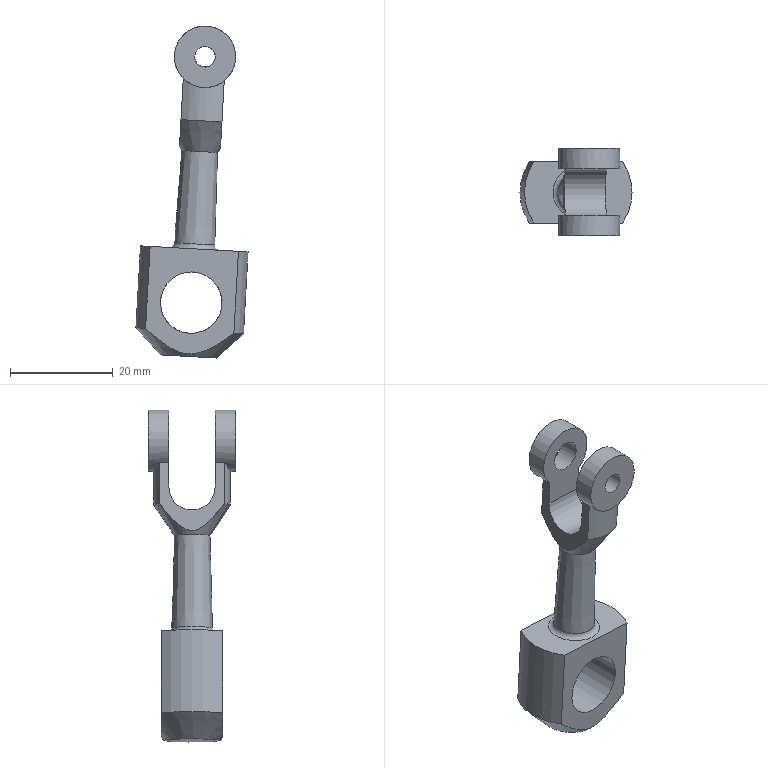Component | NX | PISTON_ROD_CONNECTING_SHAFT | 1 solid | 24 faces | volume 5624 mm3 | cylinder 10 | plane 10 | cone 3 | torus 1 | commonest cylinder face diameters 12 x3 15 x2 21 x2 9 x1 6 x1 4 x1